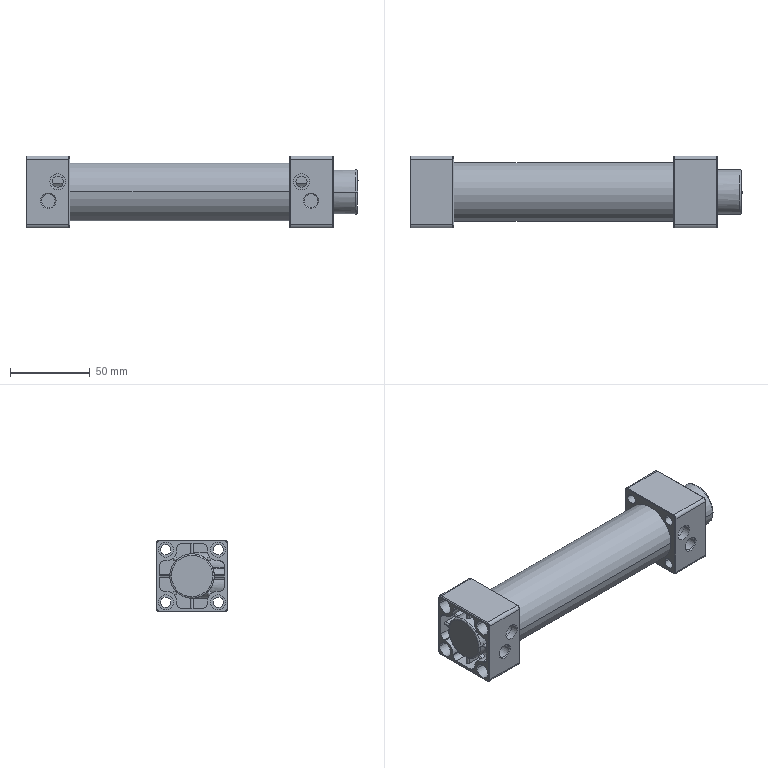Component | SolidWorks | HZ022-SC32x100S-1_HZ022-SC32x100S (1)-1 | 1 solid | 290 faces | volume 114762 mm3 | cylinder 134 | plane 122 | cone 26 | spline 8 | commonest cylinder face diameters 2 x21 6.5 x16 9.5 x16 6 x16 4 x8 14 x8 17 x5 16 x5 | material AL6061